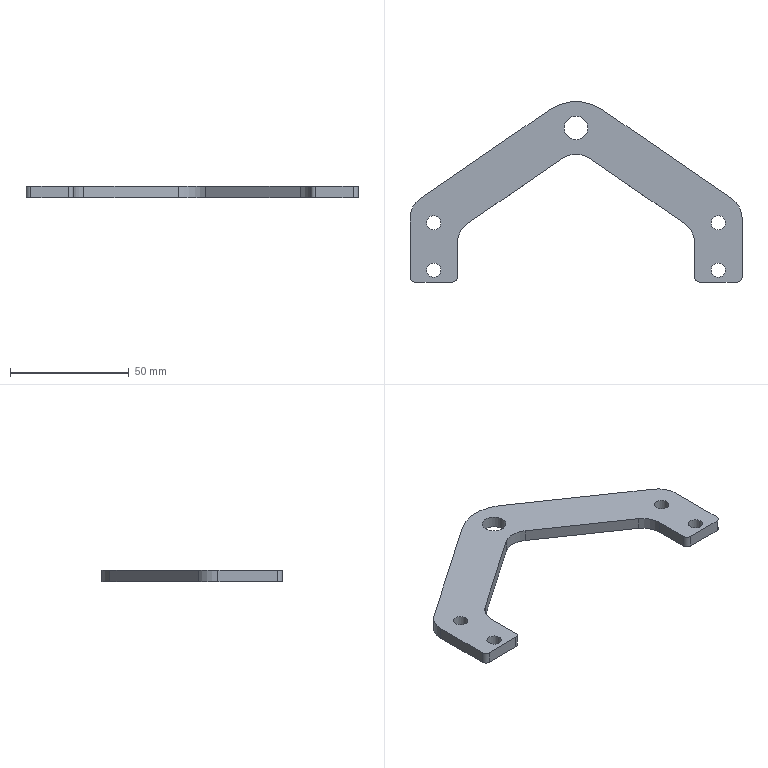Component | NX | UPPER_CONN_PLATE | 1 solid | 27 faces | volume 18853 mm3 | cylinder 15 | plane 12 | commonest cylinder face diameters 20 x5 4 x4 6 x4 10 x1 40 x1